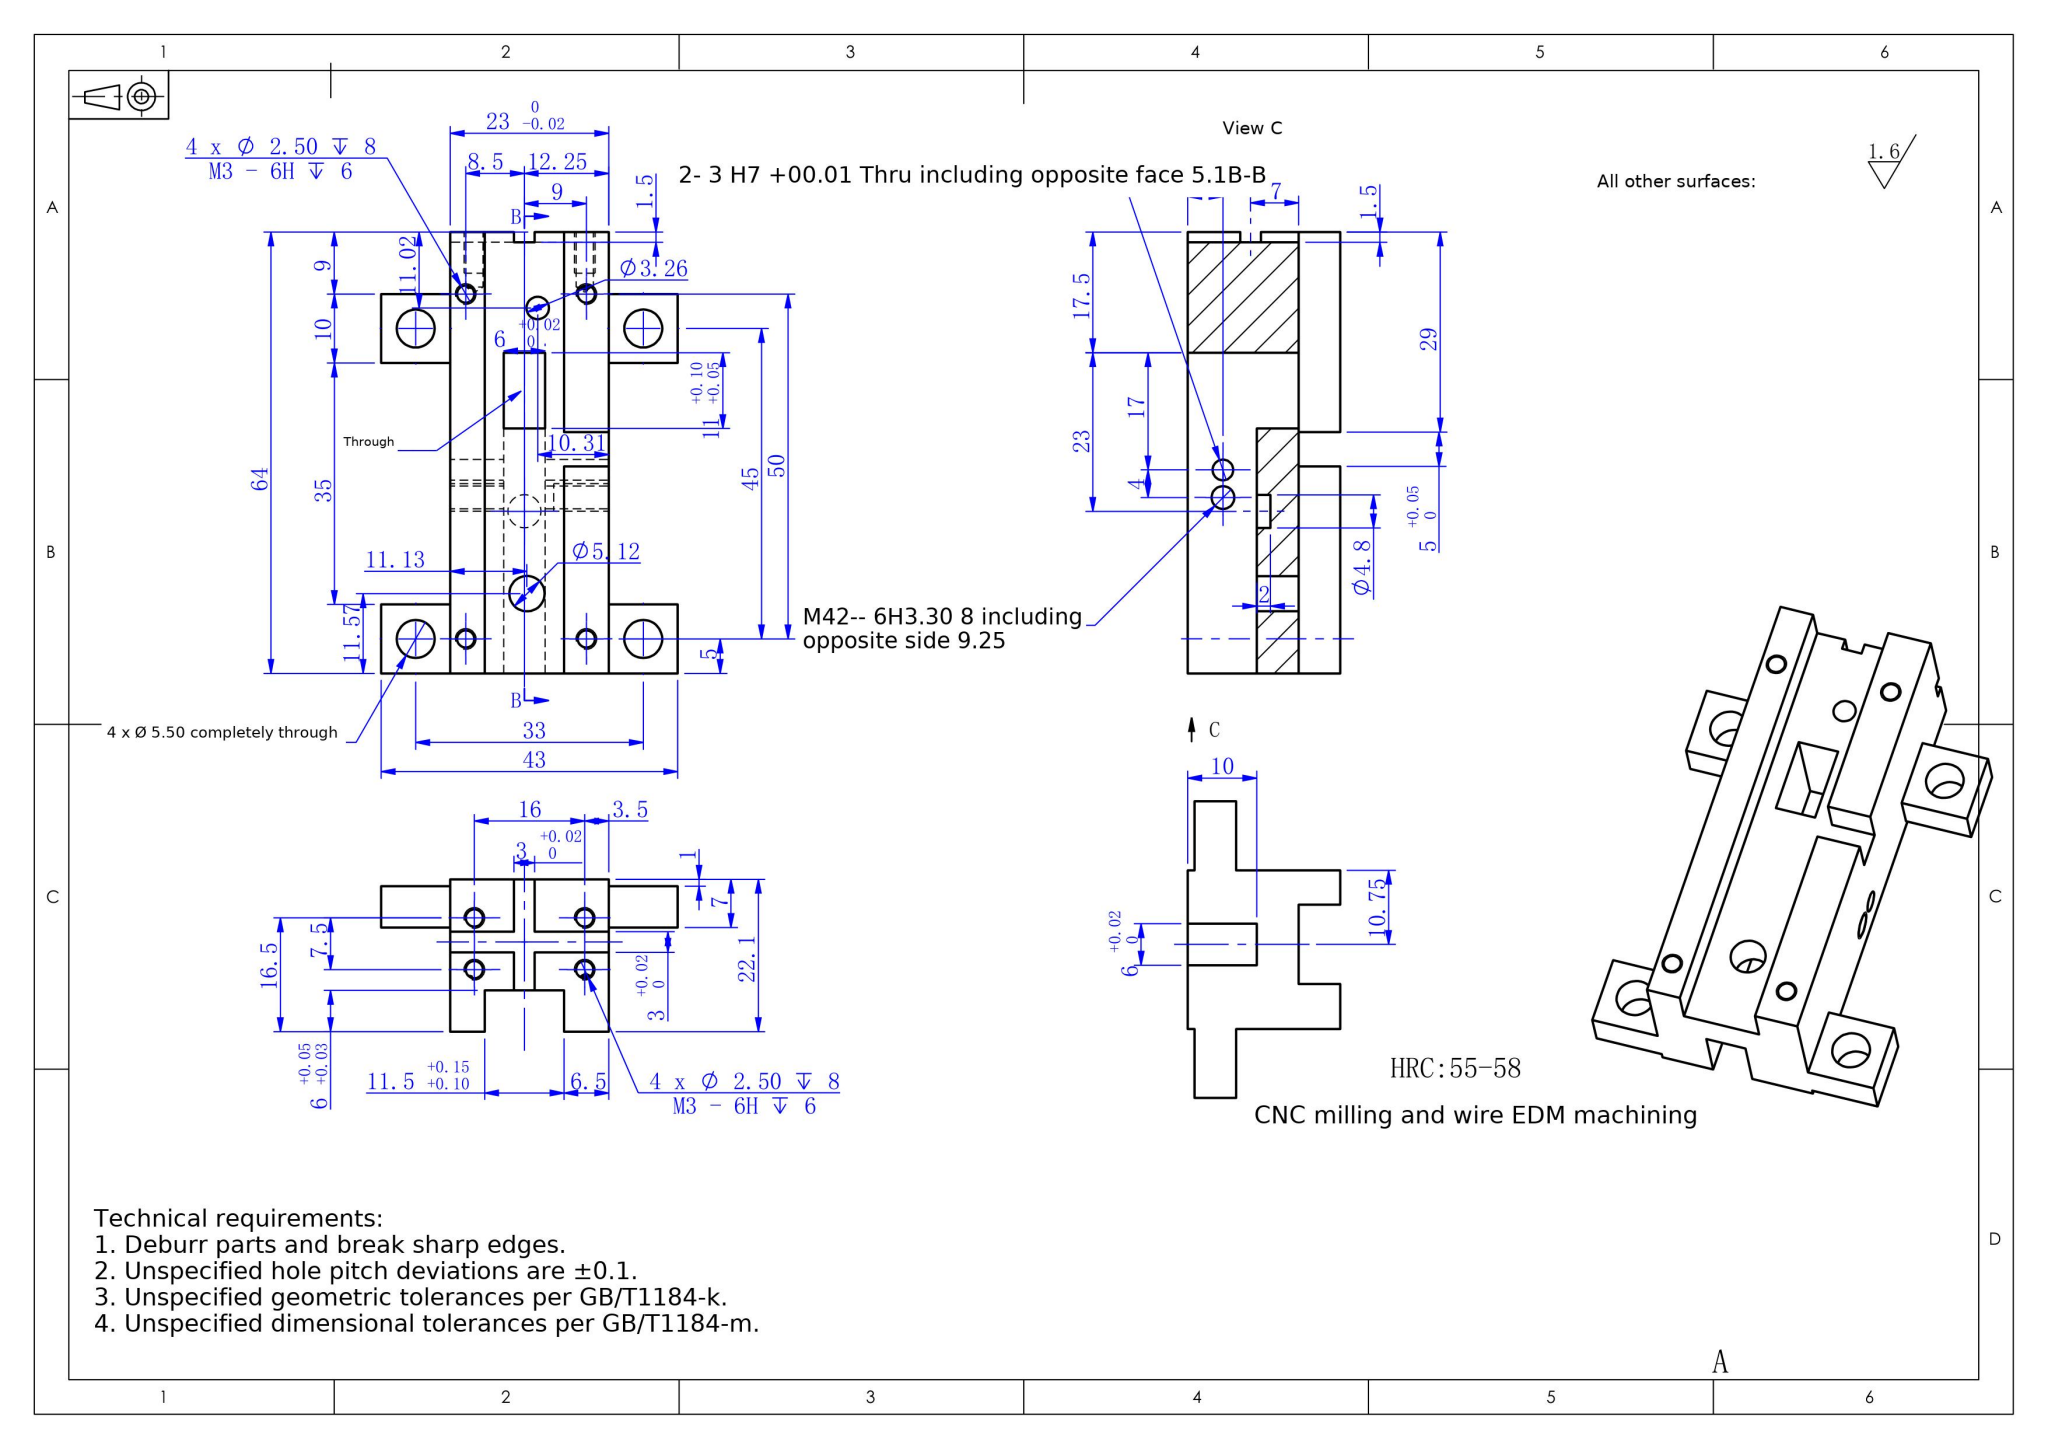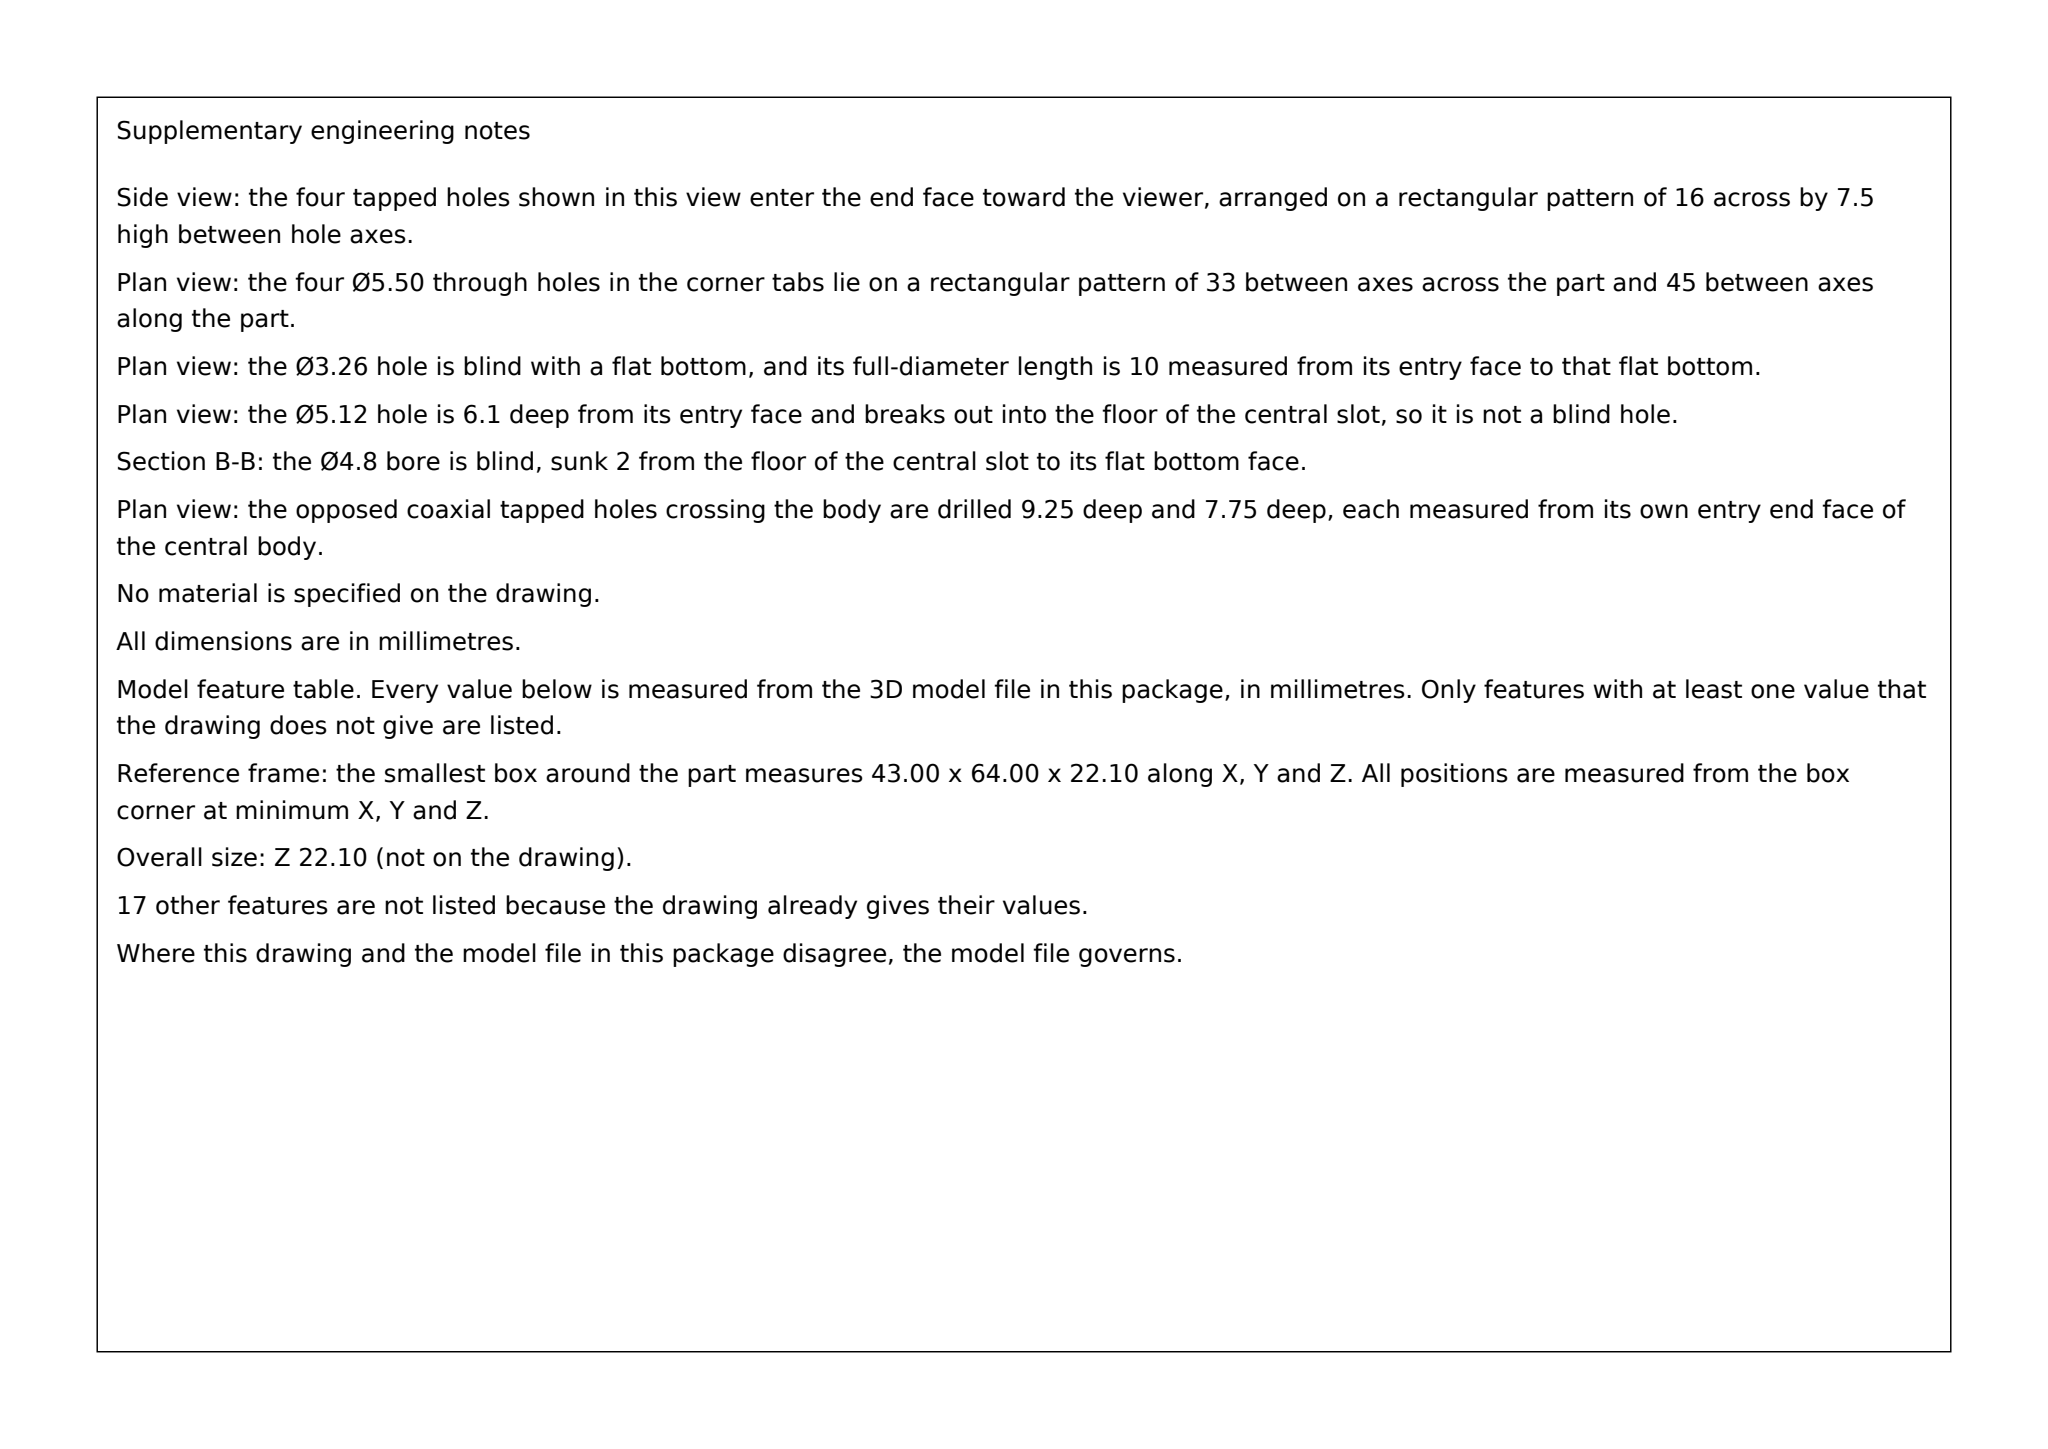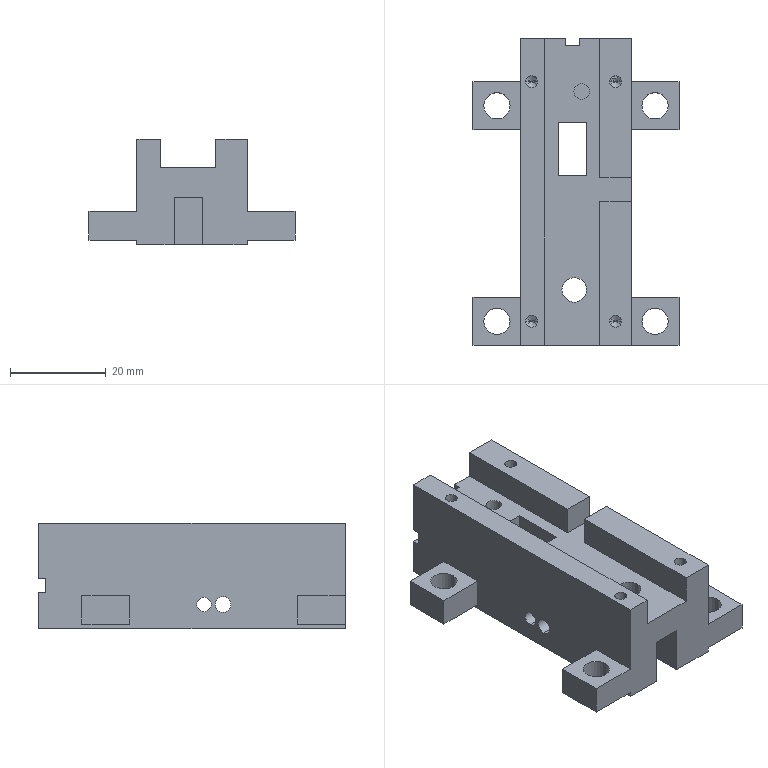Part | SolidWorks | mm | 1 solid | 105 faces | box 43 x 64 x 22.1 mm | volume 25560 mm3 | plane 51 | cylinder 38 | cone 16 | commonest cylinder face diameters 2.5 x16 5.5 x8 3.3 x4 3 x4 3.256 x2 5.12 x2 4.8 x2
Drawing notes:
Ø5.12 HOLE (FRONT VIEW, LOWER RIB): DP 6.1 | from the solid: cylinder dia 5.12, axis z, pos [21.13,11.57], length 6.1
1X Ø3.26 DP 10: X=22.69 FROM LH EDGE OF 43 (Y=52.98 FROM BOT) | from the solid: cylinder dia 3.256, axis z, pos [22.69,52.98], length 10.0
Ø4.8 DP 2 (VIEW C): X=20.75 FROM LH EDGE OF 43 | from the solid: cylinder dia 4.8, axis z, pos [20.75,23.5], length 2.0
4X Ø2.50 DP 8 / M3-6H DP 6 IN FRONT FACE: X=12.25 & 29.75 FROM LH EDGE | from the solid: cylinders dia 2.5 axis z at x=12.25 and x=29.75, y=5.0 & 55.0, length 8.0
2X Ø3 H7 THRU HOLE, AXIS PARALLEL TO X AT Y=29.5 FROM BOTTOM EDGE, Z=5.1 FROM BACK FACE; BORED 7.75 DEEP FROM ONE SIDE FACE AND 9.25 DEEP FROM OPPOSITE SIDE FACE (REPLACES GARBLED CALLOUT). | from the solid: cylinders dia 3.0, axis x, pos (y=29.5, z=5.1), lengths 7.75 and 9.25
2X M4-6H TAPPED HOLE (TAP DRILL Ø3.3), AXIS PARALLEL TO X AT Y=25.5 FROM BOTTOM EDGE, Z=5.1 FROM BACK FACE; 7.75 DEEP FROM ONE SIDE FACE AND 9.25 DEEP FROM OPPOSITE SIDE FACE (REPLACES GARBLED CALLOUT). | from the solid: cylinders dia 3.3, axis x, pos (y=25.5, z=5.1), lengths 7.75 and 9.25
6 +0.02/0 WIDE x 11 +0.10/+0.05 HIGH THRU SLOT: SLOT FLOOR AT Y=35.5 AND TOP AT Y=46.5 FROM BOTTOM EDGE OF 64; SLOT SIDES AT X=17.75 AND X=23.75 FROM LH EDGE OF 43 (CENTRED AT X=20.75). | from the solid: axis_planes y=35.5, y=46.5 and x=17.75, x=23.75
Ø5.12 HOLE DP 6.1 LOCATED X=21.13 FROM LH EDGE OF 43 AND Y=11.57 FROM BOTTOM EDGE OF 64. | from the solid: cylinder dia 5.12, axis z, pos (21.13, 11.57), length 6.1
3 +0.02/0 WIDE SLOT (TOP VIEW): SIDE FACES AT X=19.25 AND X=22.25 FROM LH EDGE OF 43, CENTRED AT X=20.75. | from the solid: axis_planes x=19.25 (2) and x=22.25 (2)
4X Ø2.50 DP 8 / M3-6H DP 6 IN SIDE FACE: AXES PARALLEL TO Y AT X=13.5 AND X=29.5 FROM LH EDGE, Z=5.6 AND Z=13.1 FROM BACK FACE. | from the solid: cylinders dia 2.5, axis y, pos (13.5/29.5, z=5.6/13.1), length 8.0
4X Ø5.50 THRU IN BASE LUGS: X=5.0 AND X=38.0 FROM LH EDGE OF 43, Y=5.0 AND Y=50.0 FROM BOTTOM EDGE OF 64. | from the solid: cylinders dia 5.5, axis z, pos (5,5)(5,50)(38,5)(38,50), length 6.0
6 +0.02/0 WIDE x 11 HIGH THRU SLOT (FRONT VIEW): LOWER FACE Y=35.5, UPPER FACE Y=46.5 FROM BOTTOM EDGE OF 64 | from the solid: axis_planes y=35.5 and y=46.5 (single faces, 11 mm apart)
2X Ø3 H7 HOLE, AXIS ALONG X AT Y=29.5 FROM BOTTOM EDGE, Z=5.1 FROM BACK FACE; DP 7.75 FROM ONE SIDE FACE AND 9.25 FROM OPPOSITE SIDE FACE | from the solid: cylinders dia 3.0 axis x at [y=29.5, z=5.1], lengths 7.75 and 9.25
2X M4-6H TAPPED HOLE (Ø3.3 TAP DRILL), AXIS ALONG X AT Y=25.5 FROM BOTTOM EDGE, Z=5.1 FROM BACK FACE; DP 7.75 FROM ONE SIDE FACE AND 9.25 FROM OPPOSITE SIDE FACE | from the solid: cylinders dia 3.3 axis x at [y=25.5, z=5.1], lengths 7.75 and 9.25
3 +0.02/0 WIDE SLOT (TOP VIEW): FACES AT Z=7.6 AND Z=10.6 FROM BACK FACE Z=0 | from the solid: axis_planes z=7.6 and z=10.6 (count 2 each, 3 mm apart)
Ø5.12 HOLE DP 6.1: X=21.13 FROM LH EDGE OF 43, Y=11.57 FROM BOTTOM EDGE OF 64 | from the solid: cylinder dia 5.12 axis z at [21.13, 11.57], length 6.1
build123d program:
from build123d import *

# Parameters (mm, degrees)
SKETCH1_W                  = 23
SKETCH1_H                  = 70
BOSS_EXTRUDE1_DEPTH        = 20.1
SKETCH2_W                  = 6
SKETCH2_H                  = 5
CUT_EXTRUDE1_DEPTH         = 18
SKETCH3_W                  = 11.5
SKETCH3_H                  = 70
CUT_EXTRUDE2_DEPTH         = 6
SKETCH4_W                  = 6
SKETCH4_H                  = 3
BOSS_EXTRUDE2_DEPTH        = 27
SKETCH5_W                  = 1.5
SKETCH5_H                  = 3
CUT_EXTRUDE3_DEPTH         = 27
SKETCH6_R                  = 2
CUT_EXTRUDE4_DEPTH         = 5
SKETCH11_W                 = 50
SKETCH11_H                 = 6
CUT_EXTRUDE5_DEPTH         = 146.916
SKETCH12_W                 = 3
SKETCH12_H                 = 1.5
CUT_EXTRUDE6_DEPTH         = 121.994
SKETCH14_W                 = 3
SKETCH14_H                 = 1.5
CUT_EXTRUDE7_DEPTH         = 65.508
M3_TAPPED_HOLE2_D          = 2.5
M3_TAPPED_HOLE2_DEPTH      = 8
M3_TAPPED_HOLE2_TIP        = 0.7511
M3_TAPPED_HOLE3_D          = 2.5
M3_TAPPED_HOLE3_DEPTH      = 8
M3_TAPPED_HOLE3_TIP        = 0.7511
BOSS_EXTRUDE3_DEPTH        = 2
SKETCH21_W                 = 6
SKETCH21_H                 = 11
CUT_EXTRUDE9_DEPTH         = 122.243
SKETCH22_W                 = 6
SKETCH22_H                 = 35.5
CUT_EXTRUDE10_DEPTH        = 10
SKETCH23_R                 = 1.5
CUT_EXTRUDE11_DEPTH        = 65.508
SKETCH24_R                 = 2.4
CUT_EXTRUDE12_DEPTH        = 2
M4_TAPPED_HOLE1_REACH      = 66.508
M4_TAPPED_HOLE1_BORE_R     = 1.65
M4_TAPPED_HOLE2_D          = 3.3
SKETCH30_W                 = 6
SKETCH30_H                 = 10
BOSS_EXTRUDE4_DEPTH        = 10
F_5_5_5_5_DIAMETER_HOLE1_D = 5.5
SKETCH35_R                 = 2.56
SKETCH35_R_2               = 1.628
CUT_EXTRUDE13_DEPTH        = 10


with BuildPart() as part:
    # Sketch1 → Boss-Extrude1 (new body)
    with BuildSketch(Plane.XY):
        with Locations((-94.388, -21.818)):
            Rectangle(SKETCH1_W, SKETCH1_H)
    extrude(amount=BOSS_EXTRUDE1_DEPTH)

    # Sketch2 → Cut-Extrude1 (cut)
    with BuildSketch(Plane(origin=(-82.888, 0, 0), x_dir=(0, 0, -1), z_dir=(1, 0, 0))):
        with Locations((-17.1, -24.318)):
            Rectangle(SKETCH2_W, SKETCH2_H)
    extrude(amount=-CUT_EXTRUDE1_DEPTH, mode=Mode.SUBTRACT)

    # Sketch3 → Cut-Extrude2 (cut)
    with BuildSketch(Plane.XY.offset(20.1)):
        with Locations((-95.138, -21.818)):
            Rectangle(SKETCH3_W, SKETCH3_H)
    extrude(amount=-CUT_EXTRUDE2_DEPTH, mode=Mode.SUBTRACT)

    # Sketch4 → Boss-Extrude2 (add)
    with BuildSketch(Plane.ZY.offset(105.888)):
        with Locations((17.1, 11.682)):
            Rectangle(SKETCH4_W, SKETCH4_H)
    extrude(amount=BOSS_EXTRUDE2_DEPTH)

    # Sketch5 → Cut-Extrude3 (cut)
    with BuildSketch(Plane.ZY.offset(132.888)):
        with Locations((19.35, 11.682)):
            Rectangle(SKETCH5_W, SKETCH5_H)
        with Locations((14.85, 11.682)):
            Rectangle(SKETCH5_W, SKETCH5_H)
    extrude(amount=-CUT_EXTRUDE3_DEPTH, mode=Mode.SUBTRACT)

    # Sketch6 → Cut-Extrude4 (cut)
    with BuildSketch(Plane.ZY.offset(132.888)):
        with Locations((17.1, 9.182)):
            Circle(SKETCH6_R)
    extrude(amount=-CUT_EXTRUDE4_DEPTH, mode=Mode.SUBTRACT)

    # Sketch11 → Cut-Extrude5 (cut, through all)
    with BuildSketch(Plane.XY.offset(20.1)):
        with Locations((-107.888, 10.182)):
            Rectangle(SKETCH11_W, SKETCH11_H)
    extrude(amount=-CUT_EXTRUDE5_DEPTH, mode=Mode.SUBTRACT)

    # Sketch12 → Cut-Extrude6 (cut, through all)
    with BuildSketch(Plane.XY.offset(14.1)):
        with Locations((-95.138, 6.432)):
            Rectangle(SKETCH12_W, SKETCH12_H)
    extrude(amount=-CUT_EXTRUDE6_DEPTH, mode=Mode.SUBTRACT)

    # Sketch14 → Cut-Extrude7 (cut, through all)
    with BuildSketch(Plane(origin=(-82.888, 0, 0), x_dir=(0, 0, -1), z_dir=(1, 0, 0))):
        with Locations((-7.1, 6.432)):
            Rectangle(SKETCH14_W, SKETCH14_H)
    extrude(amount=-CUT_EXTRUDE7_DEPTH, mode=Mode.SUBTRACT)

    # M3 Tapped Hole2
    with Locations(Plane(origin=(0, 7.182, 0), x_dir=(1, 0, 0), z_dir=(0, 1, 0))):
        with Locations((-86.388, -11.1), (-102.388, -11.1), (-102.388, -3.6), (-86.388, -3.6)):
            Hole(M3_TAPPED_HOLE2_D / 2, depth=M3_TAPPED_HOLE2_DEPTH)
            with Locations((0, 0, -(M3_TAPPED_HOLE2_DEPTH + M3_TAPPED_HOLE2_TIP / 2))):  # 118° drill point
                Cone(0, M3_TAPPED_HOLE2_D / 2, M3_TAPPED_HOLE2_TIP, mode=Mode.SUBTRACT)

    # M3 Tapped Hole3
    with Locations(Plane.XY.offset(20.1)):
        with Locations((-86.138, -1.818), (-103.638, -1.818), (-86.138, -51.818), (-103.638, -51.818)):
            Hole(M3_TAPPED_HOLE3_D / 2, depth=M3_TAPPED_HOLE3_DEPTH)
            with Locations((0, 0, -(M3_TAPPED_HOLE3_DEPTH + M3_TAPPED_HOLE3_TIP / 2))):  # 118° drill point
                Cone(0, M3_TAPPED_HOLE3_D / 2, M3_TAPPED_HOLE3_TIP, mode=Mode.SUBTRACT)

    # Sketch19 → Boss-Extrude3 (add)
    with BuildSketch(Plane(origin=(0, 0, 0), x_dir=(-1, 0, 0), z_dir=(0, 0, -1))):
        Polygon((96.638, 5.682), (93.638, 5.682), (93.638, 7.182), (82.888, 7.182), (82.888, -56.818), (105.888, -56.818), (105.888, 7.182), (96.638, 7.182), align=None)
    extrude(amount=BOSS_EXTRUDE3_DEPTH)

    # Sketch21 → Cut-Extrude9 (cut, through all)
    with BuildSketch(Plane.XY.offset(14.1)):
        with Locations((-95.138, -15.818)):
            Rectangle(SKETCH21_W, SKETCH21_H)
    extrude(amount=-CUT_EXTRUDE9_DEPTH, mode=Mode.SUBTRACT)

    # Sketch22 → Cut-Extrude10 (cut)
    with BuildSketch(Plane(origin=(0, 0, -2), x_dir=(-1, 0, 0), z_dir=(0, 0, -1))):
        with Locations((95.138, -39.068)):
            Rectangle(SKETCH22_W, SKETCH22_H)
    extrude(amount=-CUT_EXTRUDE10_DEPTH, mode=Mode.SUBTRACT)

    # Sketch23 → Cut-Extrude11 (cut, through all)
    with BuildSketch(Plane(origin=(-82.888, 0, 0), x_dir=(0, 0, -1), z_dir=(1, 0, 0))):
        with Locations((-3.1, -27.318)):
            Circle(SKETCH23_R)
    extrude(amount=-CUT_EXTRUDE11_DEPTH, mode=Mode.SUBTRACT)

    # Sketch24 → Cut-Extrude12 (cut)
    with BuildSketch(Plane(origin=(0, 0, 8), x_dir=(-1, 0, 0), z_dir=(0, 0, -1))):
        with Locations((95.138, -33.318)):
            Circle(SKETCH24_R)
    extrude(amount=-CUT_EXTRUDE12_DEPTH, mode=Mode.SUBTRACT)

    # M4 Tapped Hole1 bore → M4 Tapped Hole1 (cut, up to next)
    with BuildSketch(Plane.ZY.offset(105.888), mode=Mode.PRIVATE) as m4_tapped_hole1_sk1:
        with Locations((3.1, -31.318)):
            Circle(M4_TAPPED_HOLE1_BORE_R)
    m4_tapped_hole1_tool1 = extrude(m4_tapped_hole1_sk1.sketch, amount=-M4_TAPPED_HOLE1_REACH, mode=Mode.PRIVATE) & part.part
    add(m4_tapped_hole1_tool1.solids().sort_by_distance((-105.888, -31.318, 3.1))[0], mode=Mode.SUBTRACT)

    # M4 Tapped Hole2 (through all)
    with Locations(Plane(origin=(-82.888, 0, 0), x_dir=(0, 0, -1), z_dir=(1, 0, 0))):
        with Locations((-3.1, -31.318)):
            Hole(M4_TAPPED_HOLE2_D / 2)

    # Sketch30 → Boss-Extrude4 (add)
    with BuildSketch(Plane.ZY.offset(105.888)):
        with Locations((2, -51.818)):
            Rectangle(SKETCH30_W, SKETCH30_H)
        with Locations((2, -6.818)):
            Rectangle(SKETCH30_W, SKETCH30_H)
    boss_extrude4 = extrude(amount=BOSS_EXTRUDE4_DEPTH)

    # Mirror2: Boss-Extrude4 across plane
    add(boss_extrude4.mirror(Plane.ZY.offset(94.388)))

    # 5.5 _5.5_ Diameter Hole1 (through all)
    with Locations(Plane.XY.offset(5)):
        with Locations((-110.888, -6.818), (-110.888, -51.818)):
            f_5_5_5_5_diameter_hole1 = Hole(F_5_5_5_5_DIAMETER_HOLE1_D / 2)

    # Mirror3: 5.5 _5.5_ Diameter Hole1 across plane
    add(f_5_5_5_5_diameter_hole1.mirror(Plane.ZY.offset(94.388)), mode=Mode.SUBTRACT)

    # Sketch35 → Cut-Extrude13 (cut)
    with BuildSketch(Plane.XY.offset(14.1)):
        with Locations((-94.754, -45.251)):
            Circle(SKETCH35_R)
        with Locations((-93.2, -3.836)):
            Circle(SKETCH35_R_2)
    extrude(amount=-CUT_EXTRUDE13_DEPTH, mode=Mode.SUBTRACT)


solid = part.part